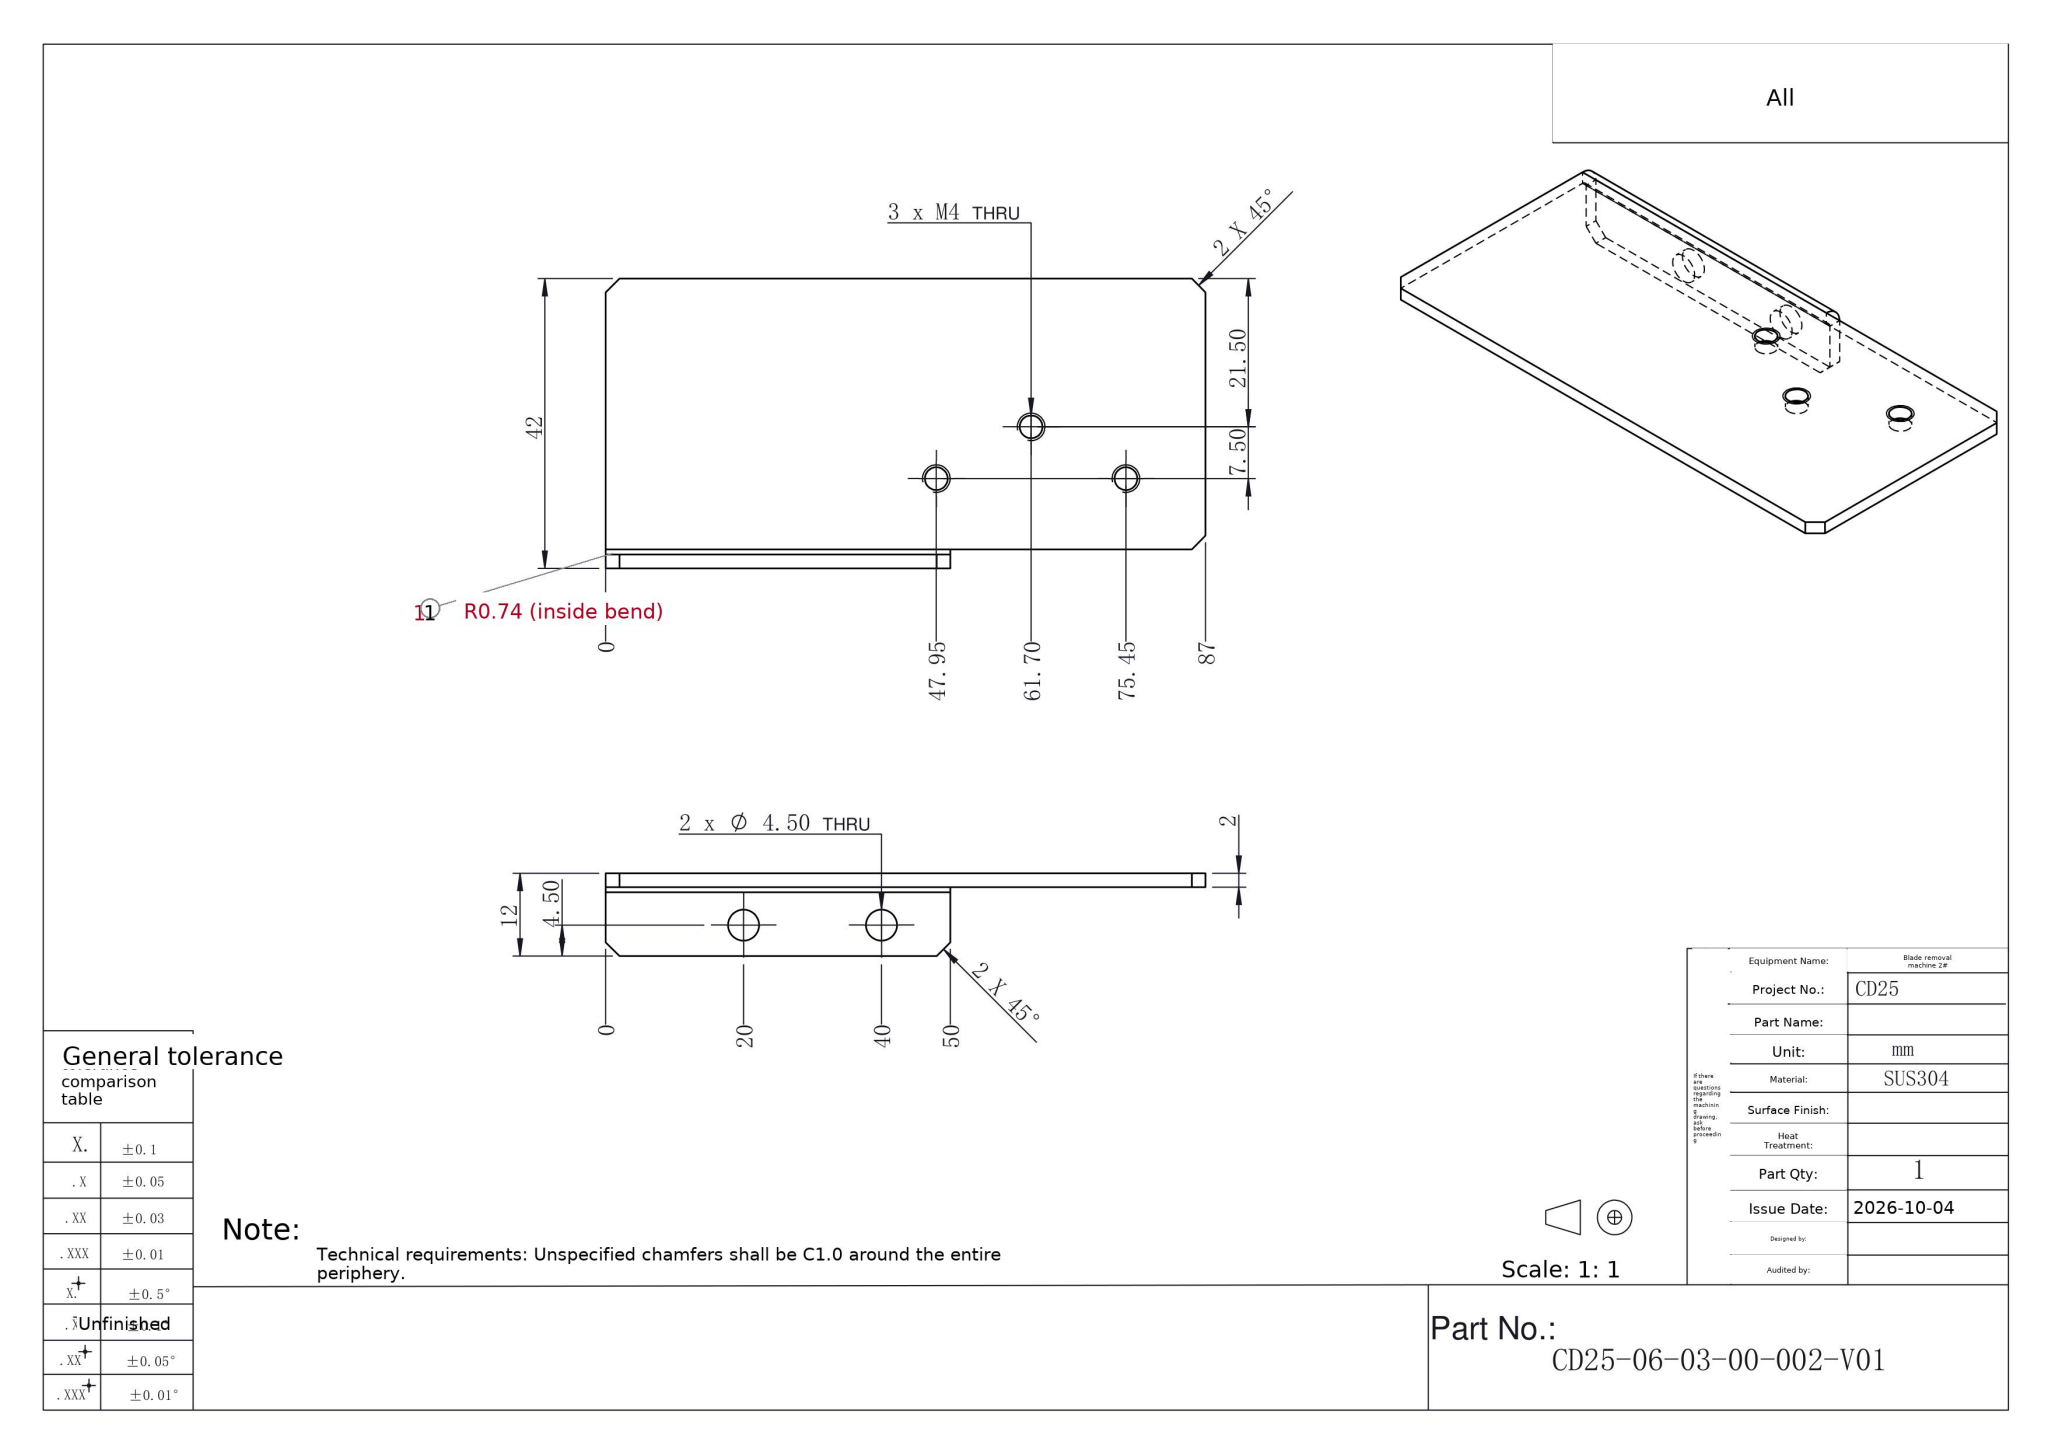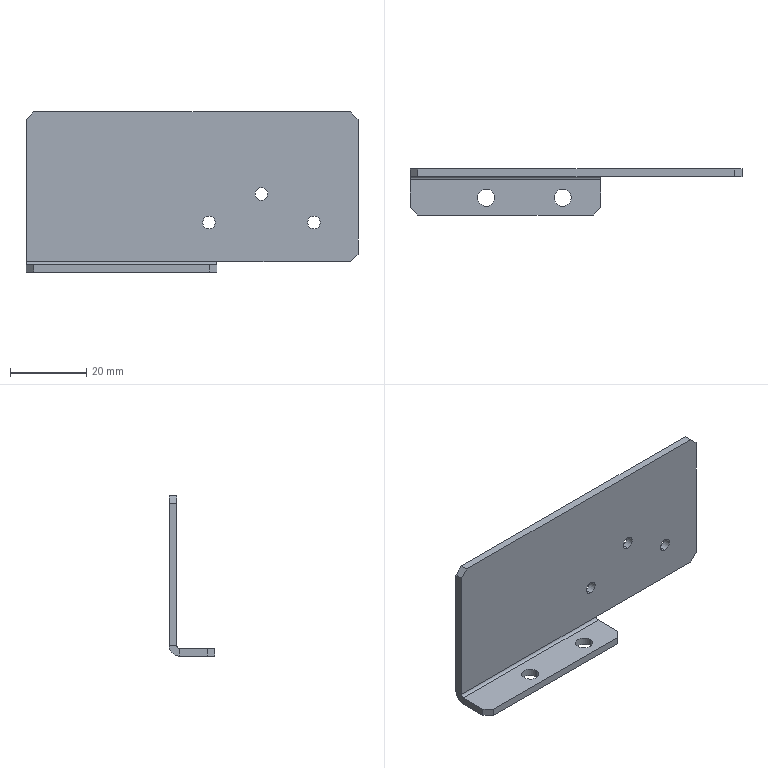Part | SolidWorks | mm | material SUS304 | 1 solid | 30 faces | box 87 x 12 x 42 mm | volume 7896 mm3 | plane 18 | cylinder 12 | commonest cylinder face diameters 3.3 x6 4.5 x4 5.473 x1 1.473 x1
STEP:
#1=CARTESIAN_POINT('',(36.7,4.,16.85));
#2=VERTEX_POINT('',#1);
#3=CARTESIAN_POINT('',(36.7,4.,20.15));
#4=VERTEX_POINT('',#3);
#5=CARTESIAN_POINT('',(36.7,4.,18.5));
#6=DIRECTION('',(0.,1.,-0.));
#7=DIRECTION('',(0.,0.,1.));
#8=AXIS2_PLACEMENT_3D('',#5,#6,#7);
#9=CIRCLE('',#8,1.65);
#10=EDGE_CURVE('',#2,#4,#9,.T.);
#11=ORIENTED_EDGE('',*,*,#10,.F.);
#12=CARTESIAN_POINT('',(36.7,6.,16.85));
#13=VERTEX_POINT('',#12);
#14=CARTESIAN_POINT('',(36.7,6.,16.85));
#15=DIRECTION('',(0.,1.,-0.));
#16=VECTOR('',#15,1000.);
#17=LINE('',#14,#16);
#18=EDGE_CURVE('',#2,#13,#17,.T.);
#19=ORIENTED_EDGE('',*,*,#18,.T.);
#20=CARTESIAN_POINT('',(36.7,6.,20.15));
#21=VERTEX_POINT('',#20);
#22=CARTESIAN_POINT('',(36.7,6.,18.5));
#23=DIRECTION('',(0.,1.,-0.));
#24=DIRECTION('',(0.,0.,1.));
#25=AXIS2_PLACEMENT_3D('',#22,#23,#24);
#26=CIRCLE('',#25,1.65);
#27=EDGE_CURVE('',#13,#21,#26,.T.);
#28=ORIENTED_EDGE('',*,*,#27,.T.);
#29=CARTESIAN_POINT('',(36.7,6.,20.15));
#30=DIRECTION('',(0.,1.,-0.));
#31=VECTOR('',#30,1000.);
#32=LINE('',#29,#31);
#33=EDGE_CURVE('',#4,#21,#32,.T.);
#34=ORIENTED_EDGE('',*,*,#33,.F.);
#35=EDGE_LOOP('',(#11,#19,#28,#34));
#36=FACE_OUTER_BOUND('',#35,.T.);
#37=CARTESIAN_POINT('',(36.7,6.,18.5));
#38=DIRECTION('',(0.,1.,-0.));
#39=DIRECTION('',(0.,0.,1.));
#40=AXIS2_PLACEMENT_3D('',#37,#38,#39);
#41=CYLINDRICAL_SURFACE('',#40,1.65);
#42=ADVANCED_FACE('',(#36),#41,.F.);
#43=CARTESIAN_POINT('',(22.95,4.,9.35));
#44=VERTEX_POINT('',#43);
#45=CARTESIAN_POINT('',(22.95,4.,12.65));
#46=VERTEX_POINT('',#45);
#47=CARTESIAN_POINT('',(22.95,4.,11.));
#48=DIRECTION('',(0.,1.,-0.));
#49=DIRECTION('',(0.,0.,1.));
#50=AXIS2_PLACEMENT_3D('',#47,#48,#49);
#51=CIRCLE('',#50,1.65);
#52=EDGE_CURVE('',#44,#46,#51,.T.);
#53=ORIENTED_EDGE('',*,*,#52,.F.);
#54=CARTESIAN_POINT('',(22.95,6.,9.35));
#55=VERTEX_POINT('',#54);
#56=CARTESIAN_POINT('',(22.95,6.,9.35));
#57=DIRECTION('',(0.,1.,-0.));
#58=VECTOR('',#57,1000.);
#59=LINE('',#56,#58);
#60=EDGE_CURVE('',#44,#55,#59,.T.);
#61=ORIENTED_EDGE('',*,*,#60,.T.);
#62=CARTESIAN_POINT('',(22.95,6.,12.65));
#63=VERTEX_POINT('',#62);
#64=CARTESIAN_POINT('',(22.95,6.,11.));
#65=DIRECTION('',(0.,1.,-0.));
#66=DIRECTION('',(0.,0.,1.));
#67=AXIS2_PLACEMENT_3D('',#64,#65,#66);
#68=CIRCLE('',#67,1.65);
#69=EDGE_CURVE('',#55,#63,#68,.T.);
#70=ORIENTED_EDGE('',*,*,#69,.T.);
#71=CARTESIAN_POINT('',(22.95,6.,12.65));
#72=DIRECTION('',(0.,1.,-0.));
#73=VECTOR('',#72,1000.);
#74=LINE('',#71,#73);
#75=EDGE_CURVE('',#46,#63,#74,.T.);
#76=ORIENTED_EDGE('',*,*,#75,.F.);
#77=EDGE_LOOP('',(#53,#61,#70,#76));
#78=FACE_OUTER_BOUND('',#77,.T.);
#79=CARTESIAN_POINT('',(22.95,6.,11.));
#80=DIRECTION('',(0.,1.,-0.));
#81=DIRECTION('',(0.,0.,1.));
#82=AXIS2_PLACEMENT_3D('',#79,#80,#81);
#83=CYLINDRICAL_SURFACE('',#82,1.65);
#84=ADVANCED_FACE('',(#78),#83,.F.);
#85=CARTESIAN_POINT('',(50.45,4.,9.35));
#86=VERTEX_POINT('',#85);
#87=CARTESIAN_POINT('',(50.45,4.,12.65));
#88=VERTEX_POINT('',#87);
#89=CARTESIAN_POINT('',(50.45,4.,11.));
#90=DIRECTION('',(0.,1.,-0.));
#91=DIRECTION('',(0.,0.,1.));
#92=AXIS2_PLACEMENT_3D('',#89,#90,#91);
#93=CIRCLE('',#92,1.65);
#94=EDGE_CURVE('',#86,#88,#93,.T.);
#95=ORIENTED_EDGE('',*,*,#94,.F.);
#96=CARTESIAN_POINT('',(50.45,6.,9.35));
#97=VERTEX_POINT('',#96);
#98=CARTESIAN_POINT('',(50.45,6.,9.35));
#99=DIRECTION('',(0.,1.,-0.));
#100=VECTOR('',#99,1000.);
#101=LINE('',#98,#100);
#102=EDGE_CURVE('',#86,#97,#101,.T.);
#103=ORIENTED_EDGE('',*,*,#102,.T.);
#104=CARTESIAN_POINT('',(50.45,6.,12.65));
#105=VERTEX_POINT('',#104);
#106=CARTESIAN_POINT('',(50.45,6.,11.));
#107=DIRECTION('',(0.,1.,-0.));
#108=DIRECTION('',(0.,0.,1.));
#109=AXIS2_PLACEMENT_3D('',#106,#107,#108);
#110=CIRCLE('',#109,1.65);
#111=EDGE_CURVE('',#97,#105,#110,.T.);
#112=ORIENTED_EDGE('',*,*,#111,.T.);
#113=CARTESIAN_POINT('',(50.45,6.,12.65));
#114=DIRECTION('',(0.,1.,-0.));
#115=VECTOR('',#114,1000.);
#116=LINE('',#113,#115);
#117=EDGE_CURVE('',#88,#105,#116,.T.);
#118=ORIENTED_EDGE('',*,*,#117,.F.);
#119=EDGE_LOOP('',(#95,#103,#112,#118));
#120=FACE_OUTER_BOUND('',#119,.T.);
#121=CARTESIAN_POINT('',(50.45,6.,11.));
#122=DIRECTION('',(0.,1.,-0.));
#123=DIRECTION('',(0.,0.,1.));
#124=AXIS2_PLACEMENT_3D('',#121,#122,#123);
#125=CYLINDRICAL_SURFACE('',#124,1.65);
#126=ADVANCED_FACE('',(#120),#125,.F.);
#127=CARTESIAN_POINT('',(-7.25,-1.5,-2.));
#128=VERTEX_POINT('',#127);
#129=CARTESIAN_POINT('',(-2.75,-1.5,-2.));
#130=VERTEX_POINT('',#129);
#131=CARTESIAN_POINT('',(-5.,-1.5,-2.));
#132=DIRECTION('',(0.,0.,1.));
#133=DIRECTION('',(1.,0.,0.));
#134=AXIS2_PLACEMENT_3D('',#131,#132,#133);
#135=CIRCLE('',#134,2.25);
#136=EDGE_CURVE('',#128,#130,#135,.T.);
#137=ORIENTED_EDGE('',*,*,#136,.F.);
#138=CARTESIAN_POINT('',(-7.25,-1.5,0.));
#139=VERTEX_POINT('',#138);
#140=CARTESIAN_POINT('',(-7.25,-1.5,0.));
#141=DIRECTION('',(0.,0.,1.));
#142=VECTOR('',#141,1000.);
#143=LINE('',#140,#142);
#144=EDGE_CURVE('',#128,#139,#143,.T.);
#145=ORIENTED_EDGE('',*,*,#144,.T.);
#146=CARTESIAN_POINT('',(-2.75,-1.5,0.));
#147=VERTEX_POINT('',#146);
#148=CARTESIAN_POINT('',(-5.,-1.5,0.));
#149=DIRECTION('',(0.,0.,1.));
#150=DIRECTION('',(1.,0.,0.));
#151=AXIS2_PLACEMENT_3D('',#148,#149,#150);
#152=CIRCLE('',#151,2.25);
#153=EDGE_CURVE('',#139,#147,#152,.T.);
#154=ORIENTED_EDGE('',*,*,#153,.T.);
#155=CARTESIAN_POINT('',(-2.75,-1.5,0.));
#156=DIRECTION('',(0.,0.,1.));
#157=VECTOR('',#156,1000.);
#158=LINE('',#155,#157);
#159=EDGE_CURVE('',#130,#147,#158,.T.);
#160=ORIENTED_EDGE('',*,*,#159,.F.);
#161=EDGE_LOOP('',(#137,#145,#154,#160));
#162=FACE_OUTER_BOUND('',#161,.T.);
#163=CARTESIAN_POINT('',(-5.,-1.5,0.));
#164=DIRECTION('',(0.,0.,1.));
#165=DIRECTION('',(1.,0.,0.));
#166=AXIS2_PLACEMENT_3D('',#163,#164,#165);
#167=CYLINDRICAL_SURFACE('',#166,2.25);
#168=ADVANCED_FACE('',(#162),#167,.F.);
#169=CARTESIAN_POINT('',(12.75,-1.5,-2.));
#170=VERTEX_POINT('',#169);
#171=CARTESIAN_POINT('',(17.25,-1.5,-2.));
#172=VERTEX_POINT('',#171);
#173=CARTESIAN_POINT('',(15.,-1.5,-2.));
#174=DIRECTION('',(0.,0.,1.));
#175=DIRECTION('',(1.,0.,0.));
#176=AXIS2_PLACEMENT_3D('',#173,#174,#175);
#177=CIRCLE('',#176,2.25);
#178=EDGE_CURVE('',#170,#172,#177,.T.);
#179=ORIENTED_EDGE('',*,*,#178,.F.);
#180=CARTESIAN_POINT('',(12.75,-1.5,0.));
#181=VERTEX_POINT('',#180);
#182=CARTESIAN_POINT('',(12.75,-1.5,0.));
#183=DIRECTION('',(0.,0.,1.));
#184=VECTOR('',#183,1000.);
#185=LINE('',#182,#184);
#186=EDGE_CURVE('',#170,#181,#185,.T.);
#187=ORIENTED_EDGE('',*,*,#186,.T.);
#188=CARTESIAN_POINT('',(17.25,-1.5,0.));
#189=VERTEX_POINT('',#188);
#190=CARTESIAN_POINT('',(15.,-1.5,0.));
#191=DIRECTION('',(0.,0.,1.));
#192=DIRECTION('',(1.,0.,0.));
#193=AXIS2_PLACEMENT_3D('',#190,#191,#192);
#194=CIRCLE('',#193,2.25);
#195=EDGE_CURVE('',#181,#189,#194,.T.);
#196=ORIENTED_EDGE('',*,*,#195,.T.);
#197=CARTESIAN_POINT('',(17.25,-1.5,0.));
#198=DIRECTION('',(0.,0.,1.));
#199=VECTOR('',#198,1000.);
#200=LINE('',#197,#199);
#201=EDGE_CURVE('',#172,#189,#200,.T.);
#202=ORIENTED_EDGE('',*,*,#201,.F.);
#203=EDGE_LOOP('',(#179,#187,#196,#202));
#204=FACE_OUTER_BOUND('',#203,.T.);
#205=CARTESIAN_POINT('',(15.,-1.5,0.));
#206=DIRECTION('',(0.,0.,1.));
#207=DIRECTION('',(1.,0.,0.));
#208=AXIS2_PLACEMENT_3D('',#205,#206,#207);
#209=CYLINDRICAL_SURFACE('',#208,2.25);
#210=ADVANCED_FACE('',(#204),#209,.F.);
#211=CARTESIAN_POINT('',(-25.,3.263,-2.));
#212=VERTEX_POINT('',#211);
#213=CARTESIAN_POINT('',(-25.,-4.,-2.));
#214=VERTEX_POINT('',#213);
#215=CARTESIAN_POINT('',(-25.,6.,-2.));
#216=DIRECTION('',(0.,-1.,0.));
#217=VECTOR('',#216,1000.);
#218=LINE('',#215,#217);
#219=EDGE_CURVE('',#212,#214,#218,.T.);
#220=ORIENTED_EDGE('',*,*,#219,.T.);
#221=CARTESIAN_POINT('',(-25.,-4.,0.));
#222=VERTEX_POINT('',#221);
#223=CARTESIAN_POINT('',(-25.,-4.,-2.));
#224=DIRECTION('',(0.,0.,1.));
#225=VECTOR('',#224,1000.);
#226=LINE('',#223,#225);
#227=EDGE_CURVE('',#214,#222,#226,.T.);
#228=ORIENTED_EDGE('',*,*,#227,.T.);
#229=CARTESIAN_POINT('',(-25.,3.263,0.));
#230=VERTEX_POINT('',#229);
#231=CARTESIAN_POINT('',(-25.,6.,0.));
#232=DIRECTION('',(0.,-1.,0.));
#233=VECTOR('',#232,1000.);
#234=LINE('',#231,#233);
#235=EDGE_CURVE('',#230,#222,#234,.T.);
#236=ORIENTED_EDGE('',*,*,#235,.F.);
#237=CARTESIAN_POINT('',(-25.,3.263,-0.));
#238=DIRECTION('',(0.,0.,-1.));
#239=VECTOR('',#238,1000.);
#240=LINE('',#237,#239);
#241=EDGE_CURVE('',#230,#212,#240,.T.);
#242=ORIENTED_EDGE('',*,*,#241,.T.);
#243=EDGE_LOOP('',(#220,#228,#236,#242));
#244=FACE_OUTER_BOUND('',#243,.T.);
#245=CARTESIAN_POINT('',(-25.,6.,-2.));
#246=DIRECTION('',(-1.,0.,0.));
#247=DIRECTION('',(0.,0.,1.));
#248=AXIS2_PLACEMENT_3D('',#245,#246,#247);
#249=PLANE('',#248);
#250=ADVANCED_FACE('',(#244),#249,.T.);
#251=CARTESIAN_POINT('',(-5.,-1.5,-2.));
#252=DIRECTION('',(0.,0.,1.));
#253=DIRECTION('',(1.,0.,0.));
#254=AXIS2_PLACEMENT_3D('',#251,#252,#253);
#255=CIRCLE('',#254,2.25);
#256=EDGE_CURVE('',#130,#128,#255,.T.);
#257=ORIENTED_EDGE('',*,*,#256,.T.);
#258=ORIENTED_EDGE('',*,*,#136,.T.);
#259=EDGE_LOOP('',(#257,#258));
#260=FACE_BOUND('',#259,.T.);
#261=CARTESIAN_POINT('',(15.,-1.5,-2.));
#262=DIRECTION('',(0.,0.,1.));
#263=DIRECTION('',(1.,0.,0.));
#264=AXIS2_PLACEMENT_3D('',#261,#262,#263);
#265=CIRCLE('',#264,2.25);
#266=EDGE_CURVE('',#172,#170,#265,.T.);
#267=ORIENTED_EDGE('',*,*,#266,.T.);
#268=ORIENTED_EDGE('',*,*,#178,.T.);
#269=EDGE_LOOP('',(#267,#268));
#270=FACE_BOUND('',#269,.T.);
#271=CARTESIAN_POINT('',(25.,-4.,-2.));
#272=VERTEX_POINT('',#271);
#273=CARTESIAN_POINT('',(25.,3.263,-2.));
#274=VERTEX_POINT('',#273);
#275=CARTESIAN_POINT('',(25.,6.,-2.));
#276=DIRECTION('',(0.,1.,0.));
#277=VECTOR('',#276,1000.);
#278=LINE('',#275,#277);
#279=EDGE_CURVE('',#272,#274,#278,.T.);
#280=ORIENTED_EDGE('',*,*,#279,.F.);
#281=CARTESIAN_POINT('',(23.,-6.,-2.));
#282=VERTEX_POINT('',#281);
#283=CARTESIAN_POINT('',(23.,-6.,-2.));
#284=DIRECTION('',(-0.7071,-0.7071,0.));
#285=VECTOR('',#284,1000.);
#286=LINE('',#283,#285);
#287=EDGE_CURVE('',#272,#282,#286,.T.);
#288=ORIENTED_EDGE('',*,*,#287,.T.);
#289=CARTESIAN_POINT('',(-23.,-6.,-2.));
#290=VERTEX_POINT('',#289);
#291=CARTESIAN_POINT('',(-25.,-6.,-2.));
#292=DIRECTION('',(1.,0.,0.));
#293=VECTOR('',#292,1000.);
#294=LINE('',#291,#293);
#295=EDGE_CURVE('',#290,#282,#294,.T.);
#296=ORIENTED_EDGE('',*,*,#295,.F.);
#297=CARTESIAN_POINT('',(-25.,-4.,-2.));
#298=DIRECTION('',(-0.7071,0.7071,0.));
#299=VECTOR('',#298,1000.);
#300=LINE('',#297,#299);
#301=EDGE_CURVE('',#290,#214,#300,.T.);
#302=ORIENTED_EDGE('',*,*,#301,.T.);
#303=ORIENTED_EDGE('',*,*,#219,.F.);
#304=CARTESIAN_POINT('',(-25.,3.263,-2.));
#305=DIRECTION('',(1.,0.,0.));
#306=VECTOR('',#305,1000.);
#307=LINE('',#304,#306);
#308=EDGE_CURVE('',#212,#274,#307,.T.);
#309=ORIENTED_EDGE('',*,*,#308,.T.);
#310=EDGE_LOOP('',(#280,#288,#296,#302,#303,#309));
#311=FACE_OUTER_BOUND('',#310,.T.);
#312=CARTESIAN_POINT('',(0.,0.,-2.));
#313=DIRECTION('',(0.,0.,1.));
#314=DIRECTION('',(1.,0.,0.));
#315=AXIS2_PLACEMENT_3D('',#312,#313,#314);
#316=PLANE('',#315);
#317=ADVANCED_FACE('',(#260,#270,#311),#316,.F.);
#318=CARTESIAN_POINT('',(-5.,-1.5,0.));
#319=DIRECTION('',(0.,0.,1.));
#320=DIRECTION('',(1.,0.,0.));
#321=AXIS2_PLACEMENT_3D('',#318,#319,#320);
#322=CIRCLE('',#321,2.25);
#323=EDGE_CURVE('',#147,#139,#322,.T.);
#324=ORIENTED_EDGE('',*,*,#323,.F.);
#325=ORIENTED_EDGE('',*,*,#153,.F.);
#326=EDGE_LOOP('',(#324,#325));
#327=FACE_BOUND('',#326,.T.);
#328=CARTESIAN_POINT('',(15.,-1.5,0.));
#329=DIRECTION('',(0.,0.,1.));
#330=DIRECTION('',(1.,0.,0.));
#331=AXIS2_PLACEMENT_3D('',#328,#329,#330);
#332=CIRCLE('',#331,2.25);
#333=EDGE_CURVE('',#189,#181,#332,.T.);
#334=ORIENTED_EDGE('',*,*,#333,.F.);
#335=ORIENTED_EDGE('',*,*,#195,.F.);
#336=EDGE_LOOP('',(#334,#335));
#337=FACE_BOUND('',#336,.T.);
#338=CARTESIAN_POINT('',(-23.,-6.,0.));
#339=VERTEX_POINT('',#338);
#340=CARTESIAN_POINT('',(23.,-6.,0.));
#341=VERTEX_POINT('',#340);
#342=CARTESIAN_POINT('',(-25.,-6.,0.));
#343=DIRECTION('',(1.,0.,0.));
#344=VECTOR('',#343,1000.);
#345=LINE('',#342,#344);
#346=EDGE_CURVE('',#339,#341,#345,.T.);
#347=ORIENTED_EDGE('',*,*,#346,.T.);
#348=CARTESIAN_POINT('',(25.,-4.,0.));
#349=VERTEX_POINT('',#348);
#350=CARTESIAN_POINT('',(14.5,-14.5,0.));
#351=DIRECTION('',(0.7071,0.7071,0.));
#352=VECTOR('',#351,1000.);
#353=LINE('',#350,#352);
#354=EDGE_CURVE('',#341,#349,#353,.T.);
#355=ORIENTED_EDGE('',*,*,#354,.T.);
#356=CARTESIAN_POINT('',(25.,3.263,0.));
#357=VERTEX_POINT('',#356);
#358=CARTESIAN_POINT('',(25.,6.,0.));
#359=DIRECTION('',(0.,1.,0.));
#360=VECTOR('',#359,1000.);
#361=LINE('',#358,#360);
#362=EDGE_CURVE('',#349,#357,#361,.T.);
#363=ORIENTED_EDGE('',*,*,#362,.T.);
#364=CARTESIAN_POINT('',(-25.,3.263,-0.));
#365=DIRECTION('',(1.,0.,0.));
#366=VECTOR('',#365,1000.);
#367=LINE('',#364,#366);
#368=EDGE_CURVE('',#230,#357,#367,.T.);
#369=ORIENTED_EDGE('',*,*,#368,.F.);
#370=ORIENTED_EDGE('',*,*,#235,.T.);
#371=CARTESIAN_POINT('',(-14.5,-14.5,0.));
#372=DIRECTION('',(0.7071,-0.7071,0.));
#373=VECTOR('',#372,1000.);
#374=LINE('',#371,#373);
#375=EDGE_CURVE('',#222,#339,#374,.T.);
#376=ORIENTED_EDGE('',*,*,#375,.T.);
#377=EDGE_LOOP('',(#347,#355,#363,#369,#370,#376));
#378=FACE_OUTER_BOUND('',#377,.T.);
#379=CARTESIAN_POINT('',(0.,0.,0.));
#380=DIRECTION('',(0.,0.,1.));
#381=DIRECTION('',(1.,0.,0.));
#382=AXIS2_PLACEMENT_3D('',#379,#380,#381);
#383=PLANE('',#382);
#384=ADVANCED_FACE('',(#327,#337,#378),#383,.T.);
#385=ORIENTED_EDGE('',*,*,#362,.F.);
#386=CARTESIAN_POINT('',(25.,-4.,-2.));
#387=DIRECTION('',(0.,0.,-1.));
#388=VECTOR('',#387,1000.);
#389=LINE('',#386,#388);
#390=EDGE_CURVE('',#349,#272,#389,.T.);
#391=ORIENTED_EDGE('',*,*,#390,.T.);
#392=ORIENTED_EDGE('',*,*,#279,.T.);
#393=CARTESIAN_POINT('',(25.,3.263,0.));
#394=DIRECTION('',(0.,0.,-1.));
#395=VECTOR('',#394,1000.);
#396=LINE('',#393,#395);
#397=EDGE_CURVE('',#357,#274,#396,.T.);
#398=ORIENTED_EDGE('',*,*,#397,.F.);
#399=EDGE_LOOP('',(#385,#391,#392,#398));
#400=FACE_OUTER_BOUND('',#399,.T.);
#401=CARTESIAN_POINT('',(25.,6.,-2.));
#402=DIRECTION('',(1.,-0.,0.));
#403=DIRECTION('',(0.,1.,0.));
#404=AXIS2_PLACEMENT_3D('',#401,#402,#403);
#405=PLANE('',#404);
#406=ADVANCED_FACE('',(#400),#405,.T.);
#407=ORIENTED_EDGE('',*,*,#295,.T.);
#408=CARTESIAN_POINT('',(23.,-6.,-2.));
#409=DIRECTION('',(0.,0.,1.));
#410=VECTOR('',#409,1000.);
#411=LINE('',#408,#410);
#412=EDGE_CURVE('',#282,#341,#411,.T.);
#413=ORIENTED_EDGE('',*,*,#412,.T.);
#414=ORIENTED_EDGE('',*,*,#346,.F.);
#415=CARTESIAN_POINT('',(-23.,-6.,-2.));
#416=DIRECTION('',(0.,0.,-1.));
#417=VECTOR('',#416,1000.);
#418=LINE('',#415,#417);
#419=EDGE_CURVE('',#339,#290,#418,.T.);
#420=ORIENTED_EDGE('',*,*,#419,.T.);
#421=EDGE_LOOP('',(#407,#413,#414,#420));
#422=FACE_OUTER_BOUND('',#421,.T.);
#423=CARTESIAN_POINT('',(-25.,-6.,-2.));
#424=DIRECTION('',(0.,-1.,0.));
#425=DIRECTION('',(0.,0.,-1.));
#426=AXIS2_PLACEMENT_3D('',#423,#424,#425);
#427=PLANE('',#426);
#428=ADVANCED_FACE('',(#422),#427,.T.);
#429=CARTESIAN_POINT('',(25.,4.,0.7366));
#430=VERTEX_POINT('',#429);
#431=CARTESIAN_POINT('',(25.,6.,0.7366));
#432=VERTEX_POINT('',#431);
#433=CARTESIAN_POINT('',(25.,4.,0.7366));
#434=DIRECTION('',(0.,1.,-0.));
#435=VECTOR('',#434,1000.);
#436=LINE('',#433,#435);
#437=EDGE_CURVE('',#430,#432,#436,.T.);
#438=ORIENTED_EDGE('',*,*,#437,.F.);
#439=CARTESIAN_POINT('',(25.,3.263,0.7366));
#440=DIRECTION('',(1.,0.,0.));
#441=DIRECTION('',(0.,0.,1.));
#442=AXIS2_PLACEMENT_3D('',#439,#440,#441);
#443=CIRCLE('',#442,0.7366);
#444=EDGE_CURVE('',#357,#430,#443,.T.);
#445=ORIENTED_EDGE('',*,*,#444,.F.);
#446=ORIENTED_EDGE('',*,*,#397,.T.);
#447=CARTESIAN_POINT('',(25.,3.263,0.7366));
#448=DIRECTION('',(1.,0.,0.));
#449=DIRECTION('',(0.,0.,1.));
#450=AXIS2_PLACEMENT_3D('',#447,#448,#449);
#451=CIRCLE('',#450,2.737);
#452=EDGE_CURVE('',#274,#432,#451,.T.);
#453=ORIENTED_EDGE('',*,*,#452,.T.);
#454=EDGE_LOOP('',(#438,#445,#446,#453));
#455=FACE_OUTER_BOUND('',#454,.T.);
#456=CARTESIAN_POINT('',(25.,3.263,0.7366));
#457=DIRECTION('',(1.,0.,0.));
#458=DIRECTION('',(0.,0.,-1.));
#459=AXIS2_PLACEMENT_3D('',#456,#457,#458);
#460=PLANE('',#459);
#461=ADVANCED_FACE('',(#455),#460,.T.);
#462=CARTESIAN_POINT('',(-25.,4.,0.7366));
#463=VERTEX_POINT('',#462);
#464=CARTESIAN_POINT('',(-25.,3.263,0.7366));
#465=DIRECTION('',(-1.,0.,-0.));
#466=DIRECTION('',(0.,0.,1.));
#467=AXIS2_PLACEMENT_3D('',#464,#465,#466);
#468=CIRCLE('',#467,0.7366);
#469=EDGE_CURVE('',#463,#230,#468,.T.);
#470=ORIENTED_EDGE('',*,*,#469,.F.);
#471=CARTESIAN_POINT('',(-25.,6.,0.7366));
#472=VERTEX_POINT('',#471);
#473=CARTESIAN_POINT('',(-25.,4.,0.7366));
#474=DIRECTION('',(0.,1.,-0.));
#475=VECTOR('',#474,1000.);
#476=LINE('',#473,#475);
#477=EDGE_CURVE('',#463,#472,#476,.T.);
#478=ORIENTED_EDGE('',*,*,#477,.T.);
#479=CARTESIAN_POINT('',(-25.,3.263,0.7366));
#480=DIRECTION('',(-1.,0.,-0.));
#481=DIRECTION('',(0.,0.,1.));
#482=AXIS2_PLACEMENT_3D('',#479,#480,#481);
#483=CIRCLE('',#482,2.737);
#484=EDGE_CURVE('',#472,#212,#483,.T.);
#485=ORIENTED_EDGE('',*,*,#484,.T.);
#486=ORIENTED_EDGE('',*,*,#241,.F.);
#487=EDGE_LOOP('',(#470,#478,#485,#486));
#488=FACE_OUTER_BOUND('',#487,.T.);
#489=CARTESIAN_POINT('',(-25.,3.263,0.7366));
#490=DIRECTION('',(1.,0.,0.));
#491=DIRECTION('',(0.,0.,-1.));
#492=AXIS2_PLACEMENT_3D('',#489,#490,#491);
#493=PLANE('',#492);
#494=ADVANCED_FACE('',(#488),#493,.F.);
#495=ORIENTED_EDGE('',*,*,#308,.F.);
#496=ORIENTED_EDGE('',*,*,#484,.F.);
#497=CARTESIAN_POINT('',(-25.,6.,0.7366));
#498=DIRECTION('',(-1.,0.,-0.));
#499=VECTOR('',#498,1000.);
#500=LINE('',#497,#499);
#501=EDGE_CURVE('',#432,#472,#500,.T.);
#502=ORIENTED_EDGE('',*,*,#501,.F.);
#503=ORIENTED_EDGE('',*,*,#452,.F.);
#504=EDGE_LOOP('',(#495,#496,#502,#503));
#505=FACE_OUTER_BOUND('',#504,.T.);
#506=CARTESIAN_POINT('',(-25.,3.263,0.7366));
#507=DIRECTION('',(-1.,0.,-0.));
#508=DIRECTION('',(0.,1.,-0.));
#509=AXIS2_PLACEMENT_3D('',#506,#507,#508);
#510=CYLINDRICAL_SURFACE('',#509,2.737);
#511=ADVANCED_FACE('',(#505),#510,.T.);
#512=ORIENTED_EDGE('',*,*,#368,.T.);
#513=ORIENTED_EDGE('',*,*,#444,.T.);
#514=CARTESIAN_POINT('',(-25.,4.,0.7366));
#515=DIRECTION('',(-1.,0.,-0.));
#516=VECTOR('',#515,1000.);
#517=LINE('',#514,#516);
#518=EDGE_CURVE('',#430,#463,#517,.T.);
#519=ORIENTED_EDGE('',*,*,#518,.T.);
#520=ORIENTED_EDGE('',*,*,#469,.T.);
#521=EDGE_LOOP('',(#512,#513,#519,#520));
#522=FACE_OUTER_BOUND('',#521,.T.);
#523=CARTESIAN_POINT('',(-25.,3.263,0.7366));
#524=DIRECTION('',(-1.,0.,-0.));
#525=DIRECTION('',(0.,1.,-0.));
#526=AXIS2_PLACEMENT_3D('',#523,#524,#525);
#527=CYLINDRICAL_SURFACE('',#526,0.7366);
#528=ADVANCED_FACE('',(#522),#527,.F.);
#529=CARTESIAN_POINT('',(-25.,4.,38.));
#530=VERTEX_POINT('',#529);
#531=CARTESIAN_POINT('',(-25.,4.,-0.));
#532=DIRECTION('',(0.,-0.,-1.));
#533=VECTOR('',#532,1000.);
#534=LINE('',#531,#533);
#535=EDGE_CURVE('',#530,#463,#534,.T.);
#536=ORIENTED_EDGE('',*,*,#535,.F.);
#537=CARTESIAN_POINT('',(-25.,6.,38.));
#538=VERTEX_POINT('',#537);
#539=CARTESIAN_POINT('',(-25.,6.,38.));
#540=DIRECTION('',(0.,1.,-0.));
#541=VECTOR('',#540,1000.);
#542=LINE('',#539,#541);
#543=EDGE_CURVE('',#530,#538,#542,.T.);
#544=ORIENTED_EDGE('',*,*,#543,.T.);
#545=CARTESIAN_POINT('',(-25.,6.,-0.));
#546=DIRECTION('',(0.,-0.,-1.));
#547=VECTOR('',#546,1000.);
#548=LINE('',#545,#547);
#549=EDGE_CURVE('',#538,#472,#548,.T.);
#550=ORIENTED_EDGE('',*,*,#549,.T.);
#551=ORIENTED_EDGE('',*,*,#477,.F.);
#552=EDGE_LOOP('',(#536,#544,#550,#551));
#553=FACE_OUTER_BOUND('',#552,.T.);
#554=CARTESIAN_POINT('',(-25.,6.,-0.));
#555=DIRECTION('',(-1.,0.,0.));
#556=DIRECTION('',(0.,0.,1.));
#557=AXIS2_PLACEMENT_3D('',#554,#555,#556);
#558=PLANE('',#557);
#559=ADVANCED_FACE('',(#553),#558,.T.);
#560=CARTESIAN_POINT('',(62.,4.,2.737));
#561=VERTEX_POINT('',#560);
#562=CARTESIAN_POINT('',(62.,4.,38.));
#563=VERTEX_POINT('',#562);
#564=CARTESIAN_POINT('',(62.,4.,-0.));
#565=DIRECTION('',(-0.,0.,1.));
#566=VECTOR('',#565,1000.);
#567=LINE('',#564,#566);
#568=EDGE_CURVE('',#561,#563,#567,.T.);
#569=ORIENTED_EDGE('',*,*,#568,.F.);
#570=CARTESIAN_POINT('',(62.,6.,2.737));
#571=VERTEX_POINT('',#570);
#572=CARTESIAN_POINT('',(62.,6.,2.737));
#573=DIRECTION('',(0.,1.,-0.));
#574=VECTOR('',#573,1000.);
#575=LINE('',#572,#574);
#576=EDGE_CURVE('',#561,#571,#575,.T.);
#577=ORIENTED_EDGE('',*,*,#576,.T.);
#578=CARTESIAN_POINT('',(62.,6.,38.));
#579=VERTEX_POINT('',#578);
#580=CARTESIAN_POINT('',(62.,6.,40.));
#581=DIRECTION('',(-0.,0.,1.));
#582=VECTOR('',#581,1000.);
#583=LINE('',#580,#582);
#584=EDGE_CURVE('',#571,#579,#583,.T.);
#585=ORIENTED_EDGE('',*,*,#584,.T.);
#586=CARTESIAN_POINT('',(62.,6.,38.));
#587=DIRECTION('',(0.,-1.,0.));
#588=VECTOR('',#587,1000.);
#589=LINE('',#586,#588);
#590=EDGE_CURVE('',#579,#563,#589,.T.);
#591=ORIENTED_EDGE('',*,*,#590,.T.);
#592=EDGE_LOOP('',(#569,#577,#585,#591));
#593=FACE_OUTER_BOUND('',#592,.T.);
#594=CARTESIAN_POINT('',(62.,6.,40.));
#595=DIRECTION('',(1.,0.,0.));
#596=DIRECTION('',(0.,0.,-1.));
#597=AXIS2_PLACEMENT_3D('',#594,#595,#596);
#598=PLANE('',#597);
#599=ADVANCED_FACE('',(#593),#598,.T.);
#600=CARTESIAN_POINT('',(36.7,6.,18.5));
#601=DIRECTION('',(0.,1.,-0.));
#602=DIRECTION('',(0.,0.,1.));
#603=AXIS2_PLACEMENT_3D('',#600,#601,#602);
#604=CIRCLE('',#603,1.65);
#605=EDGE_CURVE('',#21,#13,#604,.T.);
#606=ORIENTED_EDGE('',*,*,#605,.F.);
#607=ORIENTED_EDGE('',*,*,#27,.F.);
#608=EDGE_LOOP('',(#606,#607));
#609=FACE_BOUND('',#608,.T.);
#610=CARTESIAN_POINT('',(22.95,6.,11.));
#611=DIRECTION('',(0.,1.,-0.));
#612=DIRECTION('',(0.,0.,1.));
#613=AXIS2_PLACEMENT_3D('',#610,#611,#612);
#614=CIRCLE('',#613,1.65);
#615=EDGE_CURVE('',#63,#55,#614,.T.);
#616=ORIENTED_EDGE('',*,*,#615,.F.);
#617=ORIENTED_EDGE('',*,*,#69,.F.);
#618=EDGE_LOOP('',(#616,#617));
#619=FACE_BOUND('',#618,.T.);
#620=CARTESIAN_POINT('',(50.45,6.,11.));
#621=DIRECTION('',(0.,1.,-0.));
#622=DIRECTION('',(0.,0.,1.));
#623=AXIS2_PLACEMENT_3D('',#620,#621,#622);
#624=CIRCLE('',#623,1.65);
#625=EDGE_CURVE('',#105,#97,#624,.T.);
#626=ORIENTED_EDGE('',*,*,#625,.F.);
#627=ORIENTED_EDGE('',*,*,#111,.F.);
#628=EDGE_LOOP('',(#626,#627));
#629=FACE_BOUND('',#628,.T.);
#630=ORIENTED_EDGE('',*,*,#549,.F.);
#631=CARTESIAN_POINT('',(-23.,6.,40.));
#632=VERTEX_POINT('',#631);
#633=CARTESIAN_POINT('',(-31.5,6.,31.5));
#634=DIRECTION('',(0.7071,0.,0.7071));
#635=VECTOR('',#634,1000.);
#636=LINE('',#633,#635);
#637=EDGE_CURVE('',#538,#632,#636,.T.);
#638=ORIENTED_EDGE('',*,*,#637,.T.);
#639=CARTESIAN_POINT('',(60.,6.,40.));
#640=VERTEX_POINT('',#639);
#641=CARTESIAN_POINT('',(-25.,6.,40.));
#642=DIRECTION('',(-1.,0.,-0.));
#643=VECTOR('',#642,1000.);
#644=LINE('',#641,#643);
#645=EDGE_CURVE('',#640,#632,#644,.T.);
#646=ORIENTED_EDGE('',*,*,#645,.F.);
#647=CARTESIAN_POINT('',(50.,6.,50.));
#648=DIRECTION('',(0.7071,-0.,-0.7071));
#649=VECTOR('',#648,1000.);
#650=LINE('',#647,#649);
#651=EDGE_CURVE('',#640,#579,#650,.T.);
#652=ORIENTED_EDGE('',*,*,#651,.T.);
#653=ORIENTED_EDGE('',*,*,#584,.F.);
#654=CARTESIAN_POINT('',(60.,6.,0.7366));
#655=VERTEX_POINT('',#654);
#656=CARTESIAN_POINT('',(29.632,6.,-29.632));
#657=DIRECTION('',(-0.7071,-0.,-0.7071));
#658=VECTOR('',#657,1000.);
#659=LINE('',#656,#658);
#660=EDGE_CURVE('',#571,#655,#659,.T.);
#661=ORIENTED_EDGE('',*,*,#660,.T.);
#662=CARTESIAN_POINT('',(-0.,6.,0.7366));
#663=DIRECTION('',(-1.,-0.,-0.));
#664=VECTOR('',#663,1000.);
#665=LINE('',#662,#664);
#666=EDGE_CURVE('',#655,#432,#665,.T.);
#667=ORIENTED_EDGE('',*,*,#666,.T.);
#668=ORIENTED_EDGE('',*,*,#501,.T.);
#669=EDGE_LOOP('',(#630,#638,#646,#652,#653,#661,#667,#668));
#670=FACE_OUTER_BOUND('',#669,.T.);
#671=CARTESIAN_POINT('',(0.,6.,-0.));
#672=DIRECTION('',(0.,1.,-0.));
#673=DIRECTION('',(0.,0.,1.));
#674=AXIS2_PLACEMENT_3D('',#671,#672,#673);
#675=PLANE('',#674);
#676=ADVANCED_FACE('',(#609,#619,#629,#670),#675,.T.);
#677=CARTESIAN_POINT('',(36.7,4.,18.5));
#678=DIRECTION('',(0.,1.,-0.));
#679=DIRECTION('',(0.,0.,1.));
#680=AXIS2_PLACEMENT_3D('',#677,#678,#679);
#681=CIRCLE('',#680,1.65);
#682=EDGE_CURVE('',#4,#2,#681,.T.);
#683=ORIENTED_EDGE('',*,*,#682,.T.);
#684=ORIENTED_EDGE('',*,*,#10,.T.);
#685=EDGE_LOOP('',(#683,#684));
#686=FACE_BOUND('',#685,.T.);
#687=CARTESIAN_POINT('',(22.95,4.,11.));
#688=DIRECTION('',(0.,1.,-0.));
#689=DIRECTION('',(0.,0.,1.));
#690=AXIS2_PLACEMENT_3D('',#687,#688,#689);
#691=CIRCLE('',#690,1.65);
#692=EDGE_CURVE('',#46,#44,#691,.T.);
#693=ORIENTED_EDGE('',*,*,#692,.T.);
#694=ORIENTED_EDGE('',*,*,#52,.T.);
#695=EDGE_LOOP('',(#693,#694));
#696=FACE_BOUND('',#695,.T.);
#697=CARTESIAN_POINT('',(50.45,4.,11.));
#698=DIRECTION('',(0.,1.,-0.));
#699=DIRECTION('',(0.,0.,1.));
#700=AXIS2_PLACEMENT_3D('',#697,#698,#699);
#701=CIRCLE('',#700,1.65);
#702=EDGE_CURVE('',#88,#86,#701,.T.);
#703=ORIENTED_EDGE('',*,*,#702,.T.);
#704=ORIENTED_EDGE('',*,*,#94,.T.);
#705=EDGE_LOOP('',(#703,#704));
#706=FACE_BOUND('',#705,.T.);
#707=CARTESIAN_POINT('',(60.,4.,40.));
#708=VERTEX_POINT('',#707);
#709=CARTESIAN_POINT('',(-23.,4.,40.));
#710=VERTEX_POINT('',#709);
#711=CARTESIAN_POINT('',(0.,4.,40.));
#712=DIRECTION('',(-1.,0.,-0.));
#713=VECTOR('',#712,1000.);
#714=LINE('',#711,#713);
#715=EDGE_CURVE('',#708,#710,#714,.T.);
#716=ORIENTED_EDGE('',*,*,#715,.T.);
#717=CARTESIAN_POINT('',(-23.,4.,40.));
#718=DIRECTION('',(-0.7071,-0.,-0.7071));
#719=VECTOR('',#718,1000.);
#720=LINE('',#717,#719);
#721=EDGE_CURVE('',#710,#530,#720,.T.);
#722=ORIENTED_EDGE('',*,*,#721,.T.);
#723=ORIENTED_EDGE('',*,*,#535,.T.);
#724=ORIENTED_EDGE('',*,*,#518,.F.);
#725=CARTESIAN_POINT('',(60.,4.,0.7366));
#726=VERTEX_POINT('',#725);
#727=CARTESIAN_POINT('',(62.,4.,0.7366));
#728=DIRECTION('',(-1.,-0.,-0.));
#729=VECTOR('',#728,1000.);
#730=LINE('',#727,#729);
#731=EDGE_CURVE('',#726,#430,#730,.T.);
#732=ORIENTED_EDGE('',*,*,#731,.F.);
#733=CARTESIAN_POINT('',(62.,4.,2.737));
#734=DIRECTION('',(0.7071,0.,0.7071));
#735=VECTOR('',#734,1000.);
#736=LINE('',#733,#735);
#737=EDGE_CURVE('',#726,#561,#736,.T.);
#738=ORIENTED_EDGE('',*,*,#737,.T.);
#739=ORIENTED_EDGE('',*,*,#568,.T.);
#740=CARTESIAN_POINT('',(62.,4.,38.));
#741=DIRECTION('',(-0.7071,0.,0.7071));
#742=VECTOR('',#741,1000.);
#743=LINE('',#740,#742);
#744=EDGE_CURVE('',#563,#708,#743,.T.);
#745=ORIENTED_EDGE('',*,*,#744,.T.);
#746=EDGE_LOOP('',(#716,#722,#723,#724,#732,#738,#739,#745));
#747=FACE_OUTER_BOUND('',#746,.T.);
#748=CARTESIAN_POINT('',(0.,4.,-0.));
#749=DIRECTION('',(0.,1.,-0.));
#750=DIRECTION('',(0.,0.,1.));
#751=AXIS2_PLACEMENT_3D('',#748,#749,#750);
#752=PLANE('',#751);
#753=ADVANCED_FACE('',(#686,#696,#706,#747),#752,.F.);
#754=ORIENTED_EDGE('',*,*,#645,.T.);
#755=CARTESIAN_POINT('',(-23.,6.,40.));
#756=DIRECTION('',(0.,-1.,0.));
#757=VECTOR('',#756,1000.);
#758=LINE('',#755,#757);
#759=EDGE_CURVE('',#632,#710,#758,.T.);
#760=ORIENTED_EDGE('',*,*,#759,.T.);
#761=ORIENTED_EDGE('',*,*,#715,.F.);
#762=CARTESIAN_POINT('',(60.,6.,40.));
#763=DIRECTION('',(0.,1.,-0.));
#764=VECTOR('',#763,1000.);
#765=LINE('',#762,#764);
#766=EDGE_CURVE('',#708,#640,#765,.T.);
#767=ORIENTED_EDGE('',*,*,#766,.T.);
#768=EDGE_LOOP('',(#754,#760,#761,#767));
#769=FACE_OUTER_BOUND('',#768,.T.);
#770=CARTESIAN_POINT('',(-25.,6.,40.));
#771=DIRECTION('',(0.,0.,1.));
#772=DIRECTION('',(0.,-1.,0.));
#773=AXIS2_PLACEMENT_3D('',#770,#771,#772);
#774=PLANE('',#773);
#775=ADVANCED_FACE('',(#769),#774,.T.);
#776=ORIENTED_EDGE('',*,*,#666,.F.);
#777=CARTESIAN_POINT('',(60.,4.,0.7366));
#778=DIRECTION('',(0.,-1.,0.));
#779=VECTOR('',#778,1000.);
#780=LINE('',#777,#779);
#781=EDGE_CURVE('',#655,#726,#780,.T.);
#782=ORIENTED_EDGE('',*,*,#781,.T.);
#783=ORIENTED_EDGE('',*,*,#731,.T.);
#784=ORIENTED_EDGE('',*,*,#437,.T.);
#785=EDGE_LOOP('',(#776,#782,#783,#784));
#786=FACE_OUTER_BOUND('',#785,.T.);
#787=CARTESIAN_POINT('',(62.,4.,0.7366));
#788=DIRECTION('',(0.,-0.,-1.));
#789=DIRECTION('',(0.,1.,-0.));
#790=AXIS2_PLACEMENT_3D('',#787,#788,#789);
#791=PLANE('',#790);
#792=ADVANCED_FACE('',(#786),#791,.T.);
#793=ORIENTED_EDGE('',*,*,#287,.F.);
#794=ORIENTED_EDGE('',*,*,#390,.F.);
#795=ORIENTED_EDGE('',*,*,#354,.F.);
#796=ORIENTED_EDGE('',*,*,#412,.F.);
#797=EDGE_LOOP('',(#793,#794,#795,#796));
#798=FACE_OUTER_BOUND('',#797,.T.);
#799=CARTESIAN_POINT('',(23.,-6.,-2.));
#800=DIRECTION('',(-0.7071,0.7071,0.));
#801=DIRECTION('',(0.,0.,1.));
#802=AXIS2_PLACEMENT_3D('',#799,#800,#801);
#803=PLANE('',#802);
#804=ADVANCED_FACE('',(#798),#803,.F.);
#805=ORIENTED_EDGE('',*,*,#301,.F.);
#806=ORIENTED_EDGE('',*,*,#419,.F.);
#807=ORIENTED_EDGE('',*,*,#375,.F.);
#808=ORIENTED_EDGE('',*,*,#227,.F.);
#809=EDGE_LOOP('',(#805,#806,#807,#808));
#810=FACE_OUTER_BOUND('',#809,.T.);
#811=CARTESIAN_POINT('',(-25.,-4.,-2.));
#812=DIRECTION('',(0.7071,0.7071,0.));
#813=DIRECTION('',(0.,0.,1.));
#814=AXIS2_PLACEMENT_3D('',#811,#812,#813);
#815=PLANE('',#814);
#816=ADVANCED_FACE('',(#810),#815,.F.);
#817=ORIENTED_EDGE('',*,*,#637,.F.);
#818=ORIENTED_EDGE('',*,*,#543,.F.);
#819=ORIENTED_EDGE('',*,*,#721,.F.);
#820=ORIENTED_EDGE('',*,*,#759,.F.);
#821=EDGE_LOOP('',(#817,#818,#819,#820));
#822=FACE_OUTER_BOUND('',#821,.T.);
#823=CARTESIAN_POINT('',(-23.,6.,40.));
#824=DIRECTION('',(0.7071,-0.,-0.7071));
#825=DIRECTION('',(0.,-1.,0.));
#826=AXIS2_PLACEMENT_3D('',#823,#824,#825);
#827=PLANE('',#826);
#828=ADVANCED_FACE('',(#822),#827,.F.);
#829=ORIENTED_EDGE('',*,*,#737,.F.);
#830=ORIENTED_EDGE('',*,*,#781,.F.);
#831=ORIENTED_EDGE('',*,*,#660,.F.);
#832=ORIENTED_EDGE('',*,*,#576,.F.);
#833=EDGE_LOOP('',(#829,#830,#831,#832));
#834=FACE_OUTER_BOUND('',#833,.T.);
#835=CARTESIAN_POINT('',(62.,6.,2.737));
#836=DIRECTION('',(-0.7071,0.,0.7071));
#837=DIRECTION('',(0.,1.,-0.));
#838=AXIS2_PLACEMENT_3D('',#835,#836,#837);
#839=PLANE('',#838);
#840=ADVANCED_FACE('',(#834),#839,.F.);
#841=ORIENTED_EDGE('',*,*,#651,.F.);
#842=ORIENTED_EDGE('',*,*,#766,.F.);
#843=ORIENTED_EDGE('',*,*,#744,.F.);
#844=ORIENTED_EDGE('',*,*,#590,.F.);
#845=EDGE_LOOP('',(#841,#842,#843,#844));
#846=FACE_OUTER_BOUND('',#845,.T.);
#847=CARTESIAN_POINT('',(62.,6.,38.));
#848=DIRECTION('',(-0.7071,-0.,-0.7071));
#849=DIRECTION('',(0.,-1.,0.));
#850=AXIS2_PLACEMENT_3D('',#847,#848,#849);
#851=PLANE('',#850);
#852=ADVANCED_FACE('',(#846),#851,.F.);
#853=ORIENTED_EDGE('',*,*,#186,.F.);
#854=ORIENTED_EDGE('',*,*,#266,.F.);
#855=ORIENTED_EDGE('',*,*,#201,.T.);
#856=ORIENTED_EDGE('',*,*,#333,.T.);
#857=EDGE_LOOP('',(#853,#854,#855,#856));
#858=FACE_OUTER_BOUND('',#857,.T.);
#859=CARTESIAN_POINT('',(15.,-1.5,0.));
#860=DIRECTION('',(0.,0.,1.));
#861=DIRECTION('',(1.,0.,0.));
#862=AXIS2_PLACEMENT_3D('',#859,#860,#861);
#863=CYLINDRICAL_SURFACE('',#862,2.25);
#864=ADVANCED_FACE('',(#858),#863,.F.);
#865=ORIENTED_EDGE('',*,*,#144,.F.);
#866=ORIENTED_EDGE('',*,*,#256,.F.);
#867=ORIENTED_EDGE('',*,*,#159,.T.);
#868=ORIENTED_EDGE('',*,*,#323,.T.);
#869=EDGE_LOOP('',(#865,#866,#867,#868));
#870=FACE_OUTER_BOUND('',#869,.T.);
#871=CARTESIAN_POINT('',(-5.,-1.5,0.));
#872=DIRECTION('',(0.,0.,1.));
#873=DIRECTION('',(1.,0.,0.));
#874=AXIS2_PLACEMENT_3D('',#871,#872,#873);
#875=CYLINDRICAL_SURFACE('',#874,2.25);
#876=ADVANCED_FACE('',(#870),#875,.F.);
#877=ORIENTED_EDGE('',*,*,#102,.F.);
#878=ORIENTED_EDGE('',*,*,#702,.F.);
#879=ORIENTED_EDGE('',*,*,#117,.T.);
#880=ORIENTED_EDGE('',*,*,#625,.T.);
#881=EDGE_LOOP('',(#877,#878,#879,#880));
#882=FACE_OUTER_BOUND('',#881,.T.);
#883=CARTESIAN_POINT('',(50.45,6.,11.));
#884=DIRECTION('',(0.,1.,-0.));
#885=DIRECTION('',(0.,0.,1.));
#886=AXIS2_PLACEMENT_3D('',#883,#884,#885);
#887=CYLINDRICAL_SURFACE('',#886,1.65);
#888=ADVANCED_FACE('',(#882),#887,.F.);
#889=ORIENTED_EDGE('',*,*,#60,.F.);
#890=ORIENTED_EDGE('',*,*,#692,.F.);
#891=ORIENTED_EDGE('',*,*,#75,.T.);
#892=ORIENTED_EDGE('',*,*,#615,.T.);
#893=EDGE_LOOP('',(#889,#890,#891,#892));
#894=FACE_OUTER_BOUND('',#893,.T.);
#895=CARTESIAN_POINT('',(22.95,6.,11.));
#896=DIRECTION('',(0.,1.,-0.));
#897=DIRECTION('',(0.,0.,1.));
#898=AXIS2_PLACEMENT_3D('',#895,#896,#897);
#899=CYLINDRICAL_SURFACE('',#898,1.65);
#900=ADVANCED_FACE('',(#894),#899,.F.);
#901=ORIENTED_EDGE('',*,*,#18,.F.);
#902=ORIENTED_EDGE('',*,*,#682,.F.);
#903=ORIENTED_EDGE('',*,*,#33,.T.);
#904=ORIENTED_EDGE('',*,*,#605,.T.);
#905=EDGE_LOOP('',(#901,#902,#903,#904));
#906=FACE_OUTER_BOUND('',#905,.T.);
#907=CARTESIAN_POINT('',(36.7,6.,18.5));
#908=DIRECTION('',(0.,1.,-0.));
#909=DIRECTION('',(0.,0.,1.));
#910=AXIS2_PLACEMENT_3D('',#907,#908,#909);
#911=CYLINDRICAL_SURFACE('',#910,1.65);
#912=ADVANCED_FACE('',(#906),#911,.F.);
#913=CLOSED_SHELL('',(#42,#84,#126,#168,#210,#250,#317,#384,#406,#428,#461,#494,#511,#528,#559,#599,#676,#753,#775,#792,#804,#816,#828,#840,#852,#864,#876,#888,#900,#912));
#914=MANIFOLD_SOLID_BREP('',#913);
#915=CARTESIAN_POINT('',(0.,0.,0.));
#916=DIRECTION('',(0.,0.,1.));
#917=DIRECTION('',(1.,0.,0.));
#918=AXIS2_PLACEMENT_3D('',#915,#916,#917);
#919=(LENGTH_UNIT()NAMED_UNIT(*)SI_UNIT(.MILLI.,.METRE.));
#920=UNCERTAINTY_MEASURE_WITH_UNIT(LENGTH_MEASURE(0.00001),#919,'','');
#921=(NAMED_UNIT(*)PLANE_ANGLE_UNIT()SI_UNIT($,.RADIAN.));
#922=(NAMED_UNIT(*)SI_UNIT($,.STERADIAN.)SOLID_ANGLE_UNIT());
#923=(GEOMETRIC_REPRESENTATION_CONTEXT(3)GLOBAL_UNCERTAINTY_ASSIGNED_CONTEXT((#920))GLOBAL_UNIT_ASSIGNED_CONTEXT((#919,#921,#922))REPRESENTATION_CONTEXT('',''));
#924=ADVANCED_BREP_SHAPE_REPRESENTATION('',(#914,#918),#923);